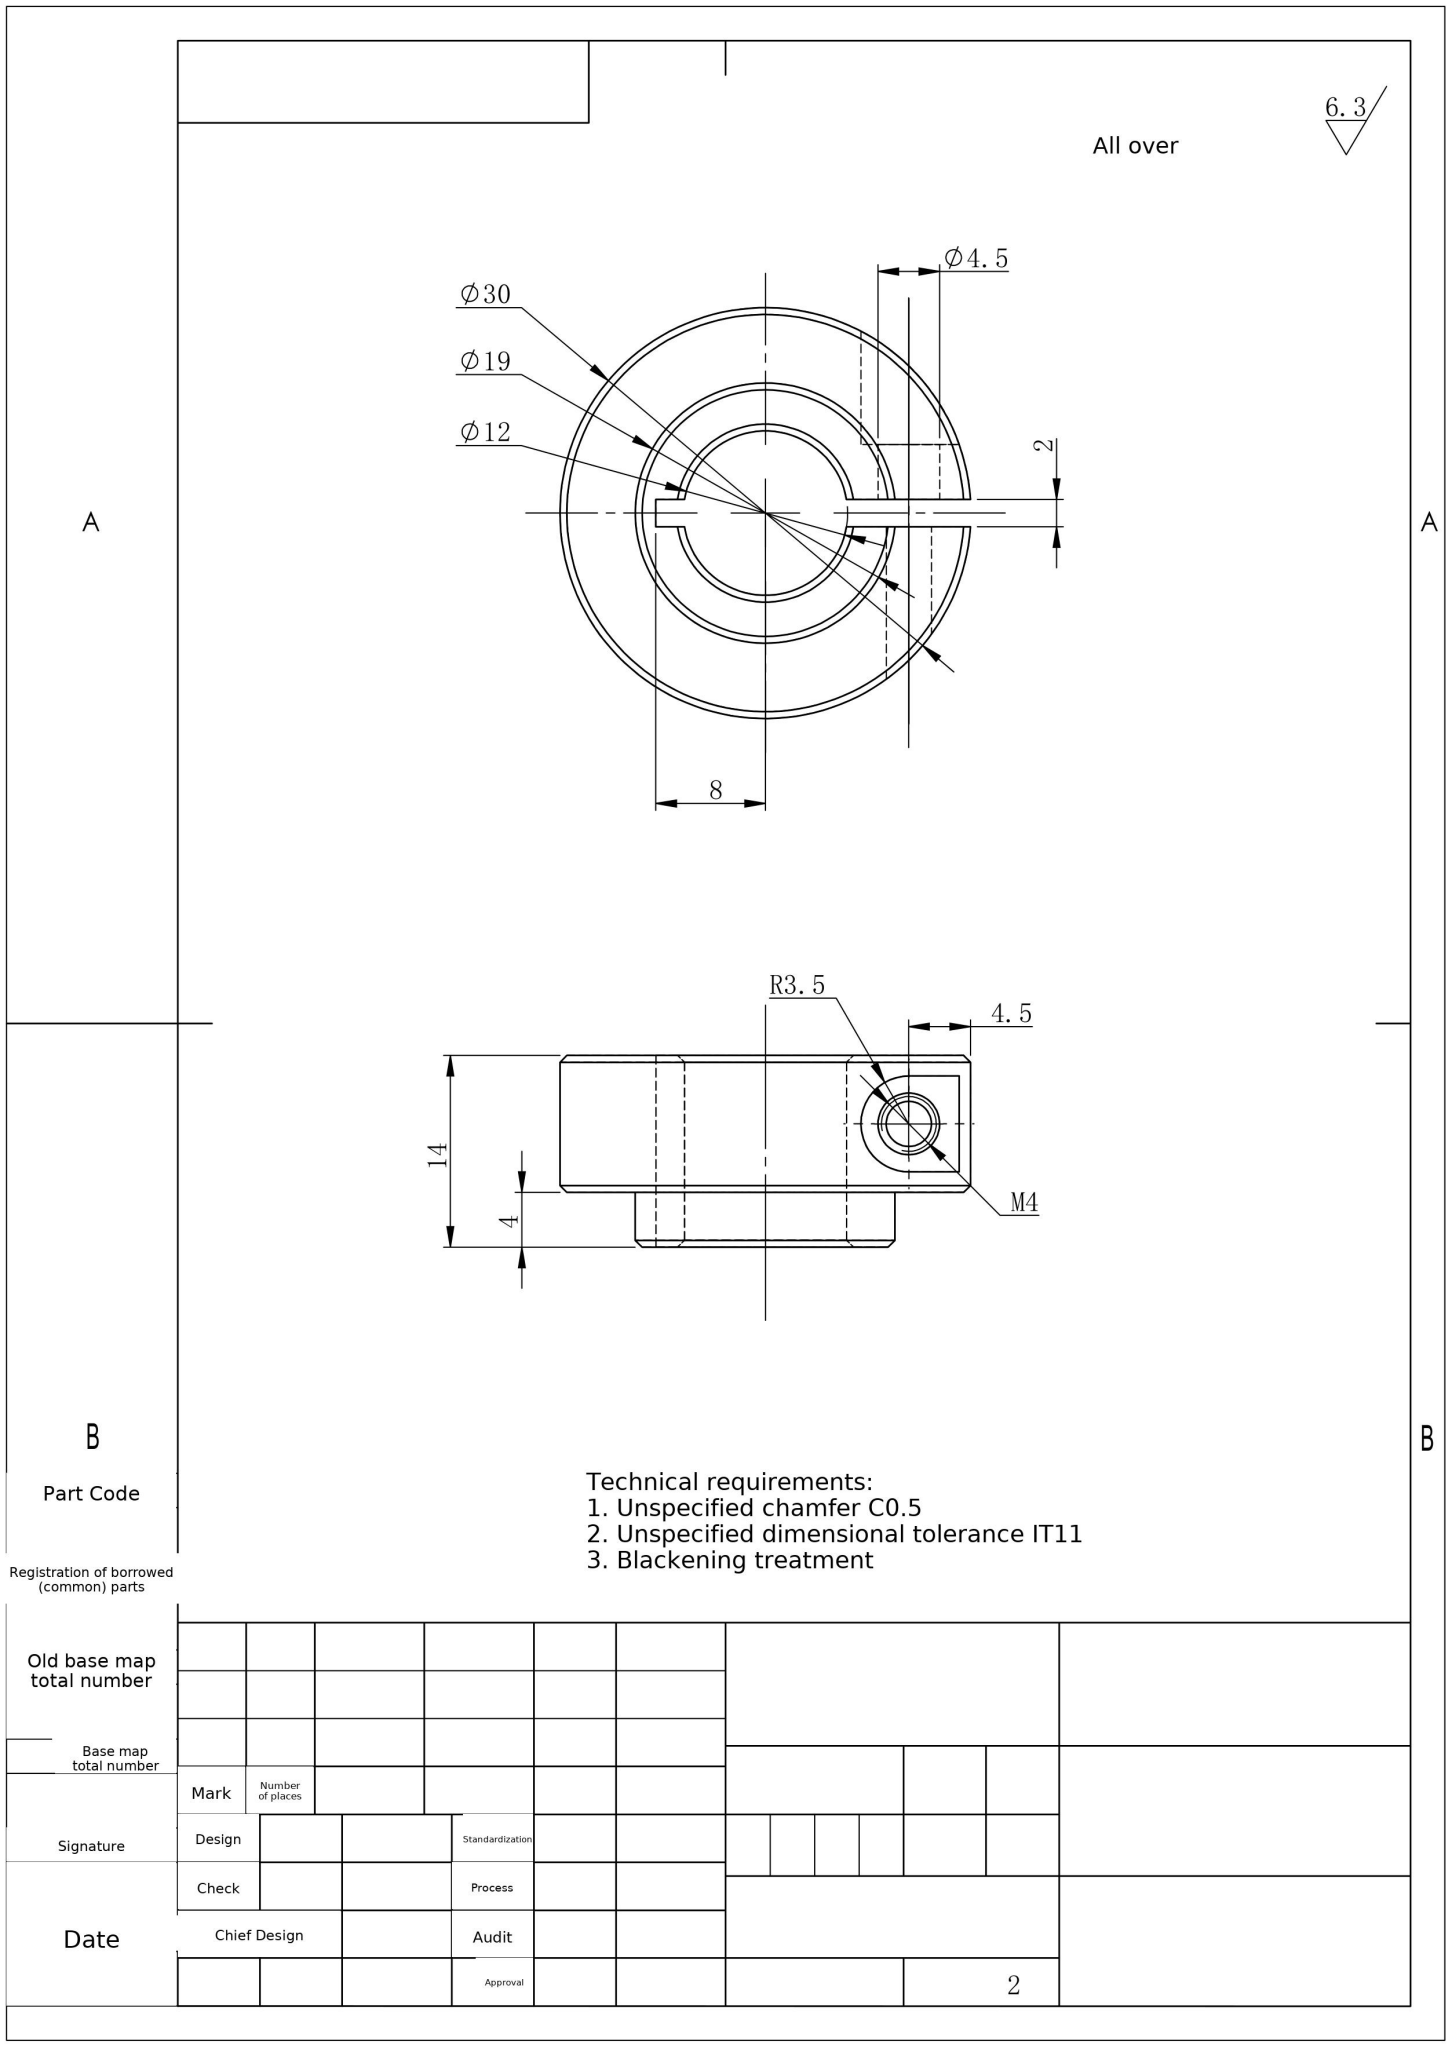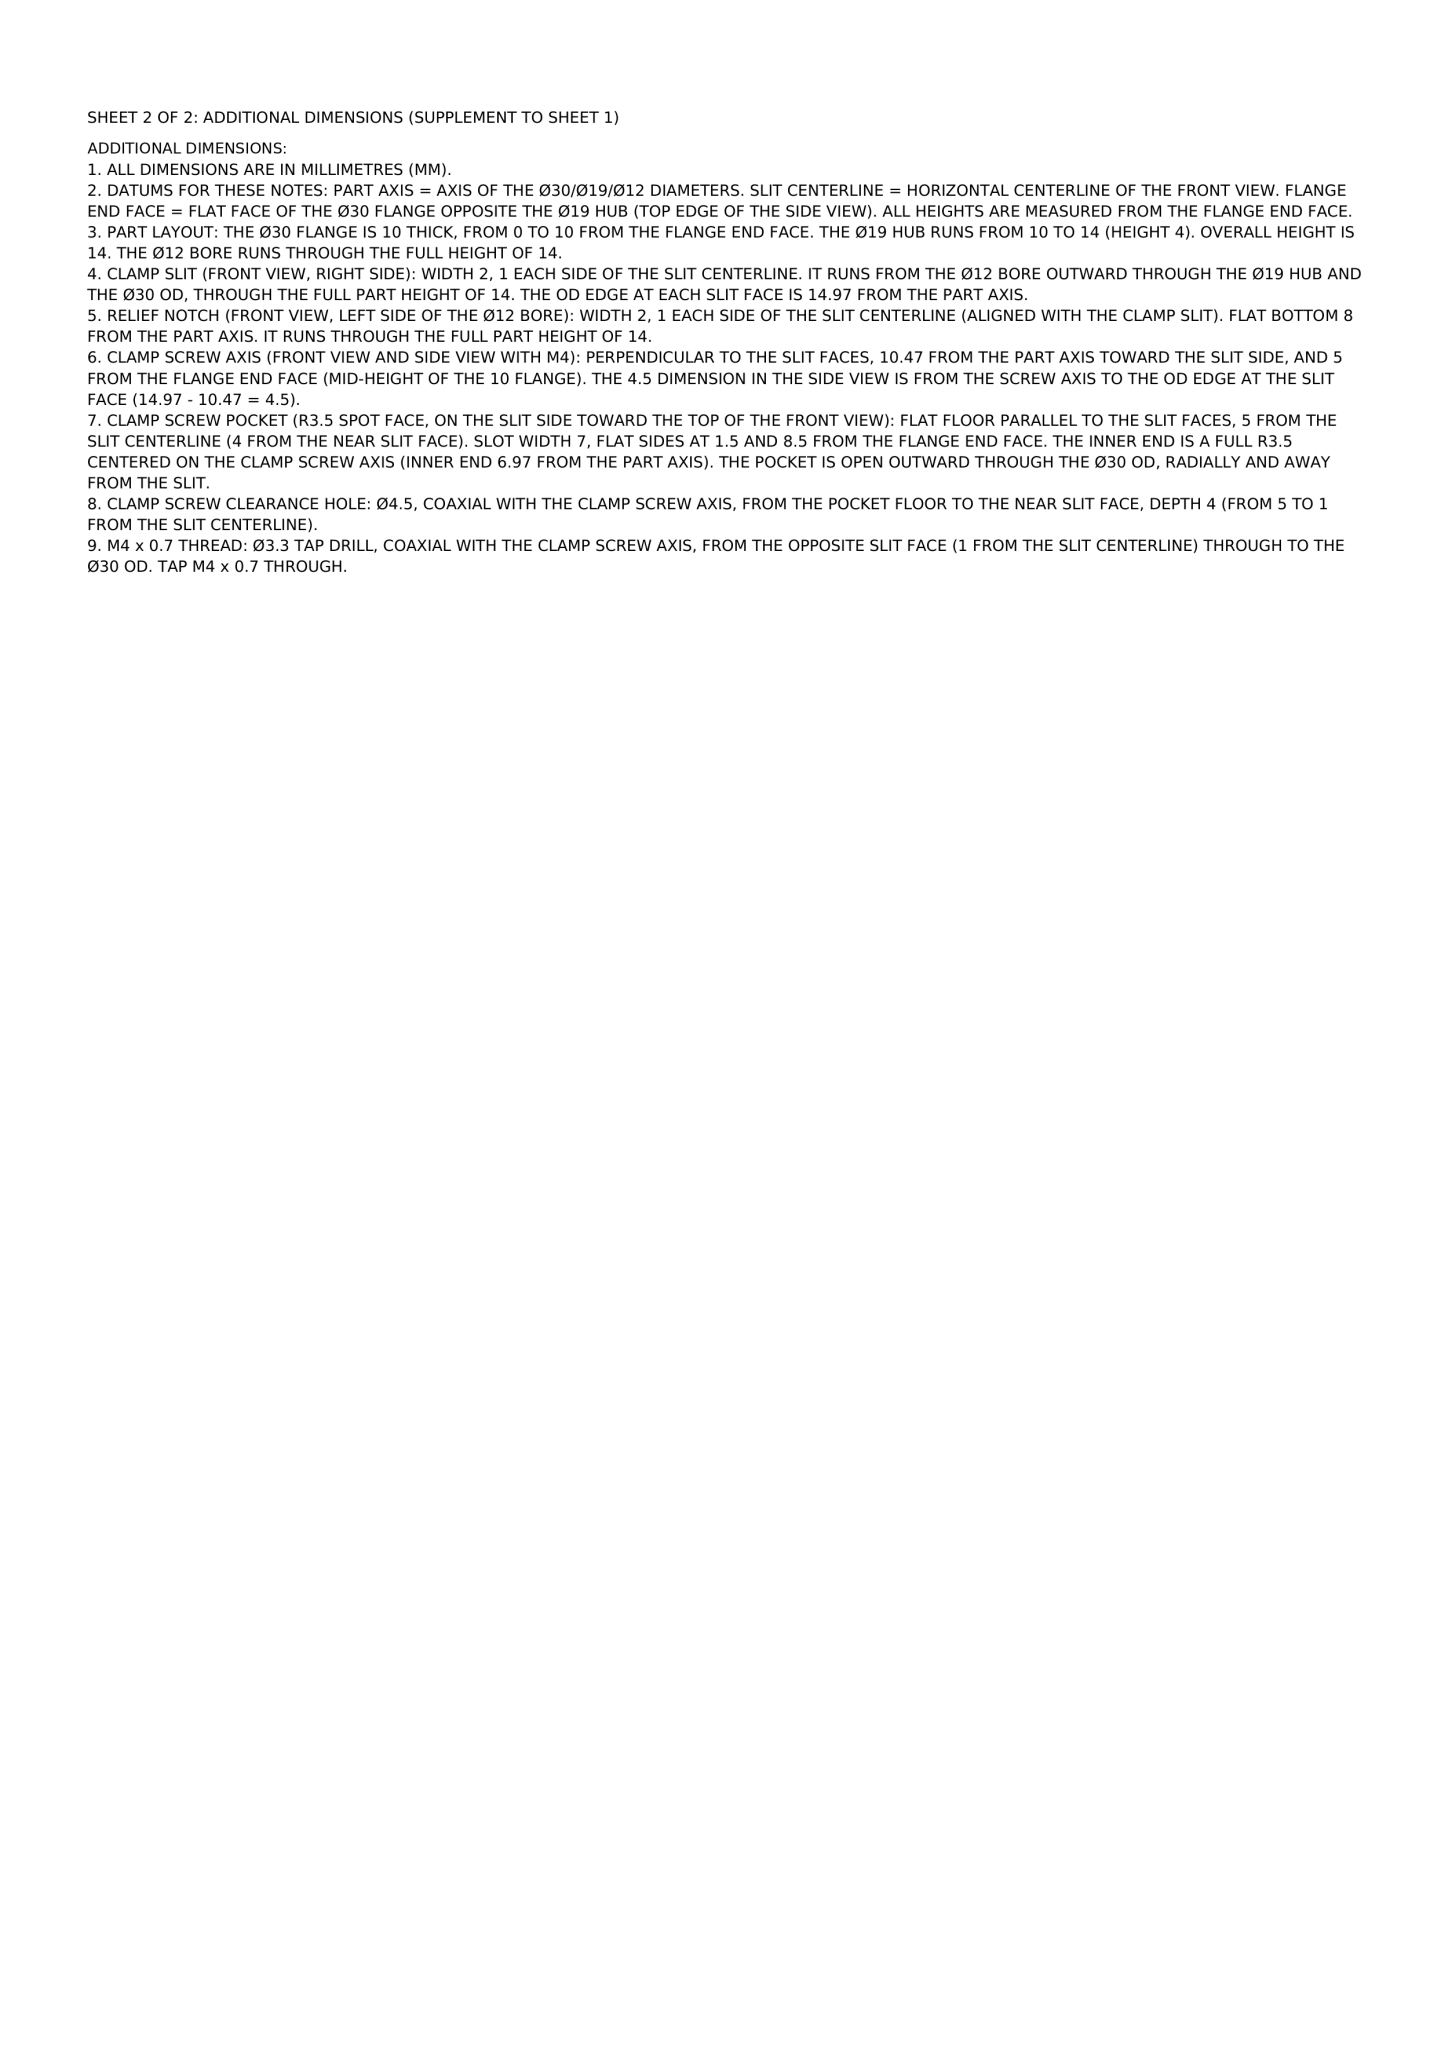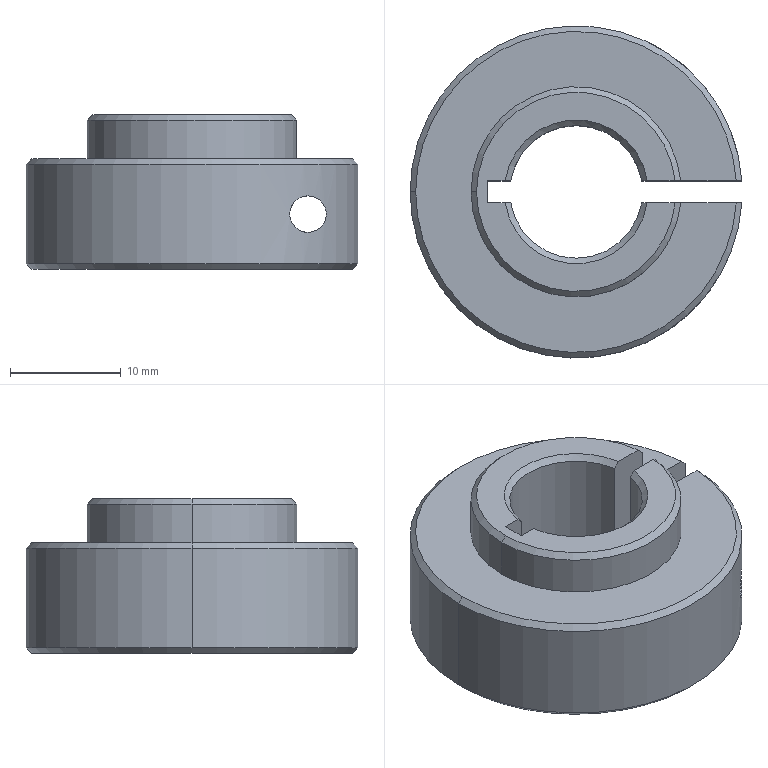Part | NX | mm | 1 solid | 31 faces | box 29.97 x 30 x 14 mm | volume 5949 mm3 | cylinder 11 | plane 11 | cone 9 | commonest cylinder face diameters 3.3 x2 19 x2 4.5 x2 30 x2 12 x2 7 x1